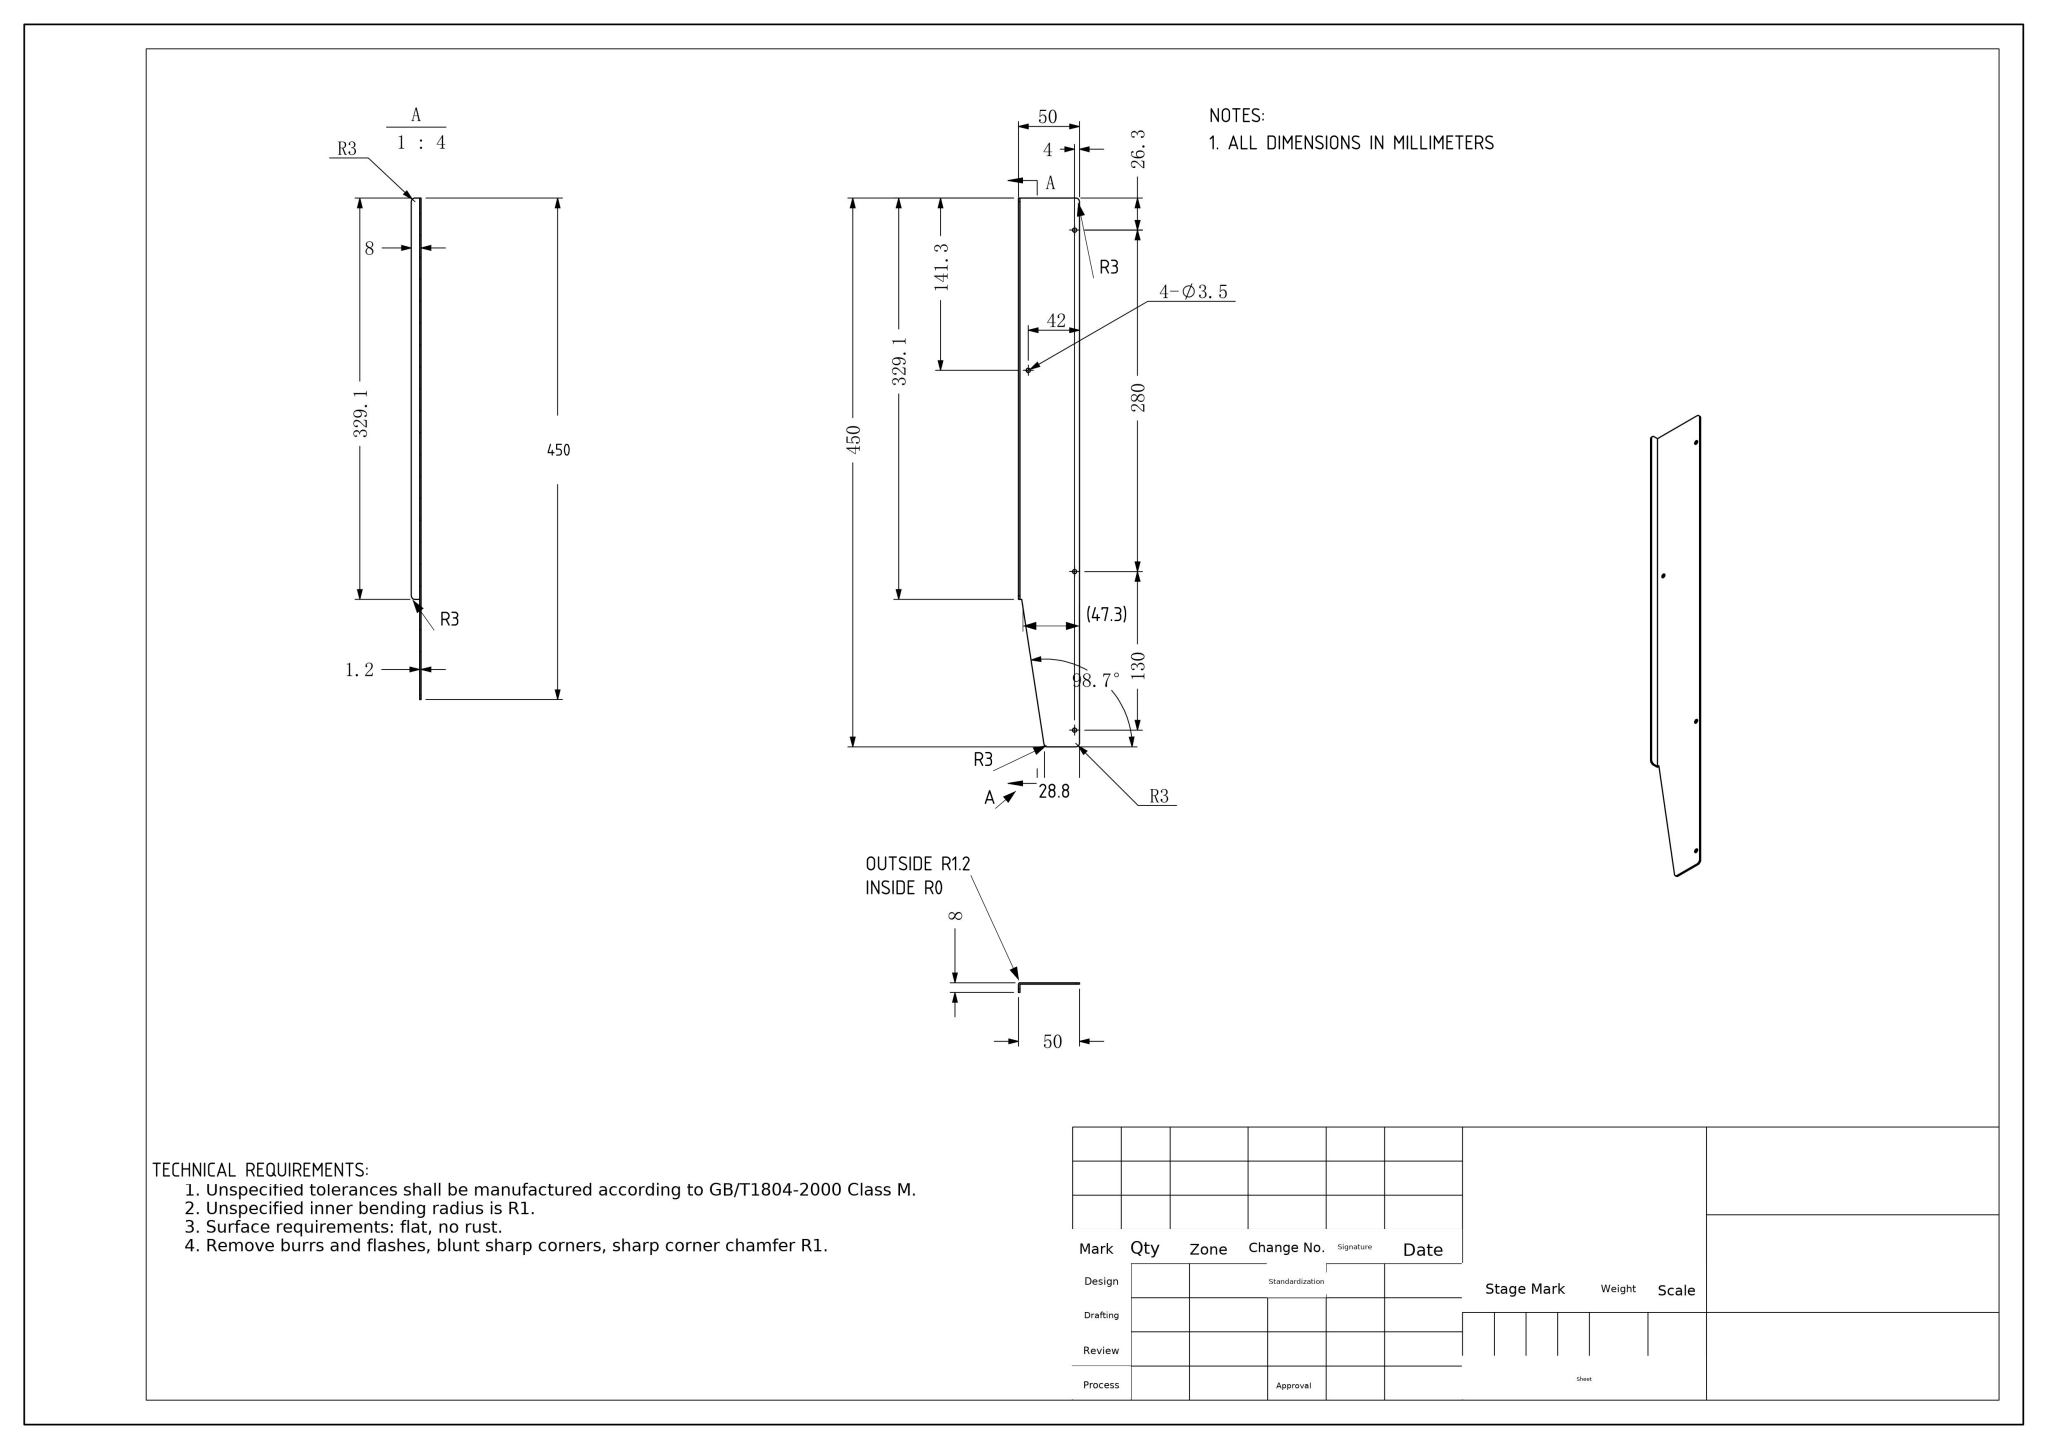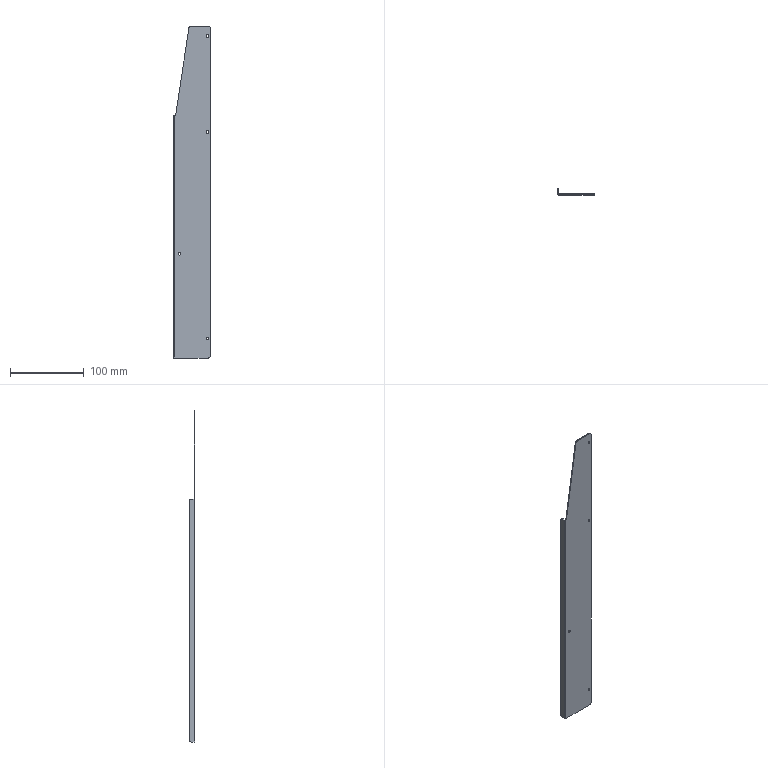Part | NX | mm | Tapered L-Shaped Shelf Bracket 329mm | 1 solid | 25 faces | box 50 x 8 x 450 mm | volume 27790 mm3 | cylinder 15 | plane 10 | commonest cylinder face diameters 3.5 x8 6 x5 2.404 x1 0.004 x1
STEP:
#1=COLOUR_RGB('',0.7529,0.7529,0.7529);
#2=FILL_AREA_STYLE_COLOUR('',#1);
#3=FILL_AREA_STYLE('',(#2));
#4=SURFACE_STYLE_FILL_AREA(#3);
#5=SURFACE_SIDE_STYLE('',(#4));
#6=SURFACE_STYLE_USAGE(.BOTH.,#5);
#7=PRESENTATION_STYLE_ASSIGNMENT((#6));
#8=CARTESIAN_POINT('',(20.,1.2,51.75));
#9=VERTEX_POINT('',#8);
#10=CARTESIAN_POINT('',(20.,1.2,48.25));
#11=VERTEX_POINT('',#10);
#12=CARTESIAN_POINT('',(20.,1.2,50.));
#13=DIRECTION('',(0.,-1.,0.));
#14=DIRECTION('',(0.,0.,-1.));
#15=AXIS2_PLACEMENT_3D('',#12,#13,#14);
#16=CIRCLE('',#15,1.75);
#17=EDGE_CURVE('',#9,#11,#16,.T.);
#18=ORIENTED_EDGE('',*,*,#17,.F.);
#19=CARTESIAN_POINT('',(20.,0.,51.75));
#20=VERTEX_POINT('',#19);
#21=CARTESIAN_POINT('',(20.,0.,51.75));
#22=DIRECTION('',(0.,-1.,0.));
#23=VECTOR('',#22,1000.);
#24=LINE('',#21,#23);
#25=EDGE_CURVE('',#9,#20,#24,.T.);
#26=ORIENTED_EDGE('',*,*,#25,.T.);
#27=CARTESIAN_POINT('',(20.,0.,48.25));
#28=VERTEX_POINT('',#27);
#29=CARTESIAN_POINT('',(20.,0.,50.));
#30=DIRECTION('',(0.,-1.,0.));
#31=DIRECTION('',(0.,0.,-1.));
#32=AXIS2_PLACEMENT_3D('',#29,#30,#31);
#33=CIRCLE('',#32,1.75);
#34=EDGE_CURVE('',#20,#28,#33,.T.);
#35=ORIENTED_EDGE('',*,*,#34,.T.);
#36=CARTESIAN_POINT('',(20.,0.,48.25));
#37=DIRECTION('',(0.,-1.,0.));
#38=VECTOR('',#37,1000.);
#39=LINE('',#36,#38);
#40=EDGE_CURVE('',#11,#28,#39,.T.);
#41=ORIENTED_EDGE('',*,*,#40,.F.);
#42=EDGE_LOOP('',(#18,#26,#35,#41));
#43=FACE_OUTER_BOUND('',#42,.T.);
#44=CARTESIAN_POINT('',(20.,0.,50.));
#45=DIRECTION('',(0.,-1.,0.));
#46=DIRECTION('',(0.,0.,-1.));
#47=AXIS2_PLACEMENT_3D('',#44,#45,#46);
#48=CYLINDRICAL_SURFACE('',#47,1.75);
#49=ADVANCED_FACE('',(#43),#48,.F.);
#50=CARTESIAN_POINT('',(20.,1.2,461.75));
#51=VERTEX_POINT('',#50);
#52=CARTESIAN_POINT('',(20.,1.2,458.25));
#53=VERTEX_POINT('',#52);
#54=CARTESIAN_POINT('',(20.,1.2,460.));
#55=DIRECTION('',(0.,-1.,0.));
#56=DIRECTION('',(0.,0.,-1.));
#57=AXIS2_PLACEMENT_3D('',#54,#55,#56);
#58=CIRCLE('',#57,1.75);
#59=EDGE_CURVE('',#51,#53,#58,.T.);
#60=ORIENTED_EDGE('',*,*,#59,.F.);
#61=CARTESIAN_POINT('',(20.,0.,461.75));
#62=VERTEX_POINT('',#61);
#63=CARTESIAN_POINT('',(20.,0.,461.75));
#64=DIRECTION('',(0.,-1.,0.));
#65=VECTOR('',#64,1000.);
#66=LINE('',#63,#65);
#67=EDGE_CURVE('',#51,#62,#66,.T.);
#68=ORIENTED_EDGE('',*,*,#67,.T.);
#69=CARTESIAN_POINT('',(20.,0.,458.25));
#70=VERTEX_POINT('',#69);
#71=CARTESIAN_POINT('',(20.,0.,460.));
#72=DIRECTION('',(0.,-1.,0.));
#73=DIRECTION('',(0.,0.,-1.));
#74=AXIS2_PLACEMENT_3D('',#71,#72,#73);
#75=CIRCLE('',#74,1.75);
#76=EDGE_CURVE('',#62,#70,#75,.T.);
#77=ORIENTED_EDGE('',*,*,#76,.T.);
#78=CARTESIAN_POINT('',(20.,0.,458.25));
#79=DIRECTION('',(0.,-1.,0.));
#80=VECTOR('',#79,1000.);
#81=LINE('',#78,#80);
#82=EDGE_CURVE('',#53,#70,#81,.T.);
#83=ORIENTED_EDGE('',*,*,#82,.F.);
#84=EDGE_LOOP('',(#60,#68,#77,#83));
#85=FACE_OUTER_BOUND('',#84,.T.);
#86=CARTESIAN_POINT('',(20.,0.,460.));
#87=DIRECTION('',(0.,-1.,0.));
#88=DIRECTION('',(0.,0.,-1.));
#89=AXIS2_PLACEMENT_3D('',#86,#87,#88);
#90=CYLINDRICAL_SURFACE('',#89,1.75);
#91=ADVANCED_FACE('',(#85),#90,.F.);
#92=CARTESIAN_POINT('',(-18.,1.2,163.25));
#93=VERTEX_POINT('',#92);
#94=CARTESIAN_POINT('',(-18.,1.2,166.75));
#95=VERTEX_POINT('',#94);
#96=CARTESIAN_POINT('',(-18.,1.2,165.));
#97=DIRECTION('',(0.,1.,0.));
#98=DIRECTION('',(0.,0.,-1.));
#99=AXIS2_PLACEMENT_3D('',#96,#97,#98);
#100=CIRCLE('',#99,1.75);
#101=EDGE_CURVE('',#93,#95,#100,.T.);
#102=ORIENTED_EDGE('',*,*,#101,.T.);
#103=CARTESIAN_POINT('',(-18.,0.,166.75));
#104=VERTEX_POINT('',#103);
#105=CARTESIAN_POINT('',(-18.,0.,166.75));
#106=DIRECTION('',(0.,-1.,0.));
#107=VECTOR('',#106,1000.);
#108=LINE('',#105,#107);
#109=EDGE_CURVE('',#95,#104,#108,.T.);
#110=ORIENTED_EDGE('',*,*,#109,.T.);
#111=CARTESIAN_POINT('',(-18.,0.,163.25));
#112=VERTEX_POINT('',#111);
#113=CARTESIAN_POINT('',(-18.,0.,165.));
#114=DIRECTION('',(0.,1.,0.));
#115=DIRECTION('',(0.,0.,-1.));
#116=AXIS2_PLACEMENT_3D('',#113,#114,#115);
#117=CIRCLE('',#116,1.75);
#118=EDGE_CURVE('',#112,#104,#117,.T.);
#119=ORIENTED_EDGE('',*,*,#118,.F.);
#120=CARTESIAN_POINT('',(-18.,0.,163.25));
#121=DIRECTION('',(0.,-1.,0.));
#122=VECTOR('',#121,1000.);
#123=LINE('',#120,#122);
#124=EDGE_CURVE('',#93,#112,#123,.T.);
#125=ORIENTED_EDGE('',*,*,#124,.F.);
#126=EDGE_LOOP('',(#102,#110,#119,#125));
#127=FACE_OUTER_BOUND('',#126,.T.);
#128=CARTESIAN_POINT('',(-18.,0.,165.));
#129=DIRECTION('',(0.,-1.,0.));
#130=DIRECTION('',(0.,0.,-1.));
#131=AXIS2_PLACEMENT_3D('',#128,#129,#130);
#132=CYLINDRICAL_SURFACE('',#131,1.75);
#133=ADVANCED_FACE('',(#127),#132,.F.);
#134=CARTESIAN_POINT('',(20.,1.2,331.75));
#135=VERTEX_POINT('',#134);
#136=CARTESIAN_POINT('',(20.,1.2,328.25));
#137=VERTEX_POINT('',#136);
#138=CARTESIAN_POINT('',(20.,1.2,330.));
#139=DIRECTION('',(0.,-1.,0.));
#140=DIRECTION('',(0.,0.,-1.));
#141=AXIS2_PLACEMENT_3D('',#138,#139,#140);
#142=CIRCLE('',#141,1.75);
#143=EDGE_CURVE('',#135,#137,#142,.T.);
#144=ORIENTED_EDGE('',*,*,#143,.F.);
#145=CARTESIAN_POINT('',(20.,0.,331.75));
#146=VERTEX_POINT('',#145);
#147=CARTESIAN_POINT('',(20.,0.,331.75));
#148=DIRECTION('',(0.,-1.,0.));
#149=VECTOR('',#148,1000.);
#150=LINE('',#147,#149);
#151=EDGE_CURVE('',#135,#146,#150,.T.);
#152=ORIENTED_EDGE('',*,*,#151,.T.);
#153=CARTESIAN_POINT('',(20.,0.,328.25));
#154=VERTEX_POINT('',#153);
#155=CARTESIAN_POINT('',(20.,0.,330.));
#156=DIRECTION('',(0.,-1.,0.));
#157=DIRECTION('',(0.,0.,-1.));
#158=AXIS2_PLACEMENT_3D('',#155,#156,#157);
#159=CIRCLE('',#158,1.75);
#160=EDGE_CURVE('',#146,#154,#159,.T.);
#161=ORIENTED_EDGE('',*,*,#160,.T.);
#162=CARTESIAN_POINT('',(20.,0.,328.25));
#163=DIRECTION('',(0.,-1.,0.));
#164=VECTOR('',#163,1000.);
#165=LINE('',#162,#164);
#166=EDGE_CURVE('',#137,#154,#165,.T.);
#167=ORIENTED_EDGE('',*,*,#166,.F.);
#168=EDGE_LOOP('',(#144,#152,#161,#167));
#169=FACE_OUTER_BOUND('',#168,.T.);
#170=CARTESIAN_POINT('',(20.,0.,330.));
#171=DIRECTION('',(0.,-1.,0.));
#172=DIRECTION('',(0.,0.,-1.));
#173=AXIS2_PLACEMENT_3D('',#170,#171,#172);
#174=CYLINDRICAL_SURFACE('',#173,1.75);
#175=ADVANCED_FACE('',(#169),#174,.F.);
#176=CARTESIAN_POINT('',(-24.8,8.,26.703));
#177=VERTEX_POINT('',#176);
#178=CARTESIAN_POINT('',(-24.8,8.,349.8));
#179=VERTEX_POINT('',#178);
#180=CARTESIAN_POINT('',(-24.8,8.,-352.8));
#181=DIRECTION('',(0.,0.,1.));
#182=VECTOR('',#181,1000.);
#183=LINE('',#180,#182);
#184=EDGE_CURVE('',#177,#179,#183,.T.);
#185=ORIENTED_EDGE('',*,*,#184,.F.);
#186=CARTESIAN_POINT('',(-26.,8.,26.703));
#187=VERTEX_POINT('',#186);
#188=CARTESIAN_POINT('',(-25.5,8.,26.703));
#189=DIRECTION('',(-1.,0.,0.));
#190=VECTOR('',#189,1000.);
#191=LINE('',#188,#190);
#192=EDGE_CURVE('',#177,#187,#191,.T.);
#193=ORIENTED_EDGE('',*,*,#192,.T.);
#194=CARTESIAN_POINT('',(-26.,8.,349.8));
#195=VERTEX_POINT('',#194);
#196=CARTESIAN_POINT('',(-26.,8.,-352.8));
#197=DIRECTION('',(0.,0.,1.));
#198=VECTOR('',#197,1000.);
#199=LINE('',#196,#198);
#200=EDGE_CURVE('',#187,#195,#199,.T.);
#201=ORIENTED_EDGE('',*,*,#200,.T.);
#202=CARTESIAN_POINT('',(-25.5,8.,349.8));
#203=DIRECTION('',(1.,0.,0.));
#204=VECTOR('',#203,1000.);
#205=LINE('',#202,#204);
#206=EDGE_CURVE('',#195,#179,#205,.T.);
#207=ORIENTED_EDGE('',*,*,#206,.T.);
#208=EDGE_LOOP('',(#185,#193,#201,#207));
#209=FACE_OUTER_BOUND('',#208,.T.);
#210=CARTESIAN_POINT('',(-25.5,8.,-352.8));
#211=DIRECTION('',(0.,-1.,0.));
#212=DIRECTION('',(0.,0.,1.));
#213=AXIS2_PLACEMENT_3D('',#210,#211,#212);
#214=PLANE('',#213);
#215=ADVANCED_FACE('',(#209),#214,.F.);
#216=CARTESIAN_POINT('',(24.,0.,26.703));
#217=VERTEX_POINT('',#216);
#218=CARTESIAN_POINT('',(24.,0.,470.703));
#219=VERTEX_POINT('',#218);
#220=CARTESIAN_POINT('',(24.,0.,-352.8));
#221=DIRECTION('',(0.,0.,1.));
#222=VECTOR('',#221,1000.);
#223=LINE('',#220,#222);
#224=EDGE_CURVE('',#217,#219,#223,.T.);
#225=ORIENTED_EDGE('',*,*,#224,.F.);
#226=CARTESIAN_POINT('',(24.,1.2,26.703));
#227=VERTEX_POINT('',#226);
#228=CARTESIAN_POINT('',(24.,1.2,26.703));
#229=DIRECTION('',(0.,1.,0.));
#230=VECTOR('',#229,1000.);
#231=LINE('',#228,#230);
#232=EDGE_CURVE('',#217,#227,#231,.T.);
#233=ORIENTED_EDGE('',*,*,#232,.T.);
#234=CARTESIAN_POINT('',(24.,1.2,470.703));
#235=VERTEX_POINT('',#234);
#236=CARTESIAN_POINT('',(24.,1.2,-352.8));
#237=DIRECTION('',(0.,0.,1.));
#238=VECTOR('',#237,1000.);
#239=LINE('',#236,#238);
#240=EDGE_CURVE('',#227,#235,#239,.T.);
#241=ORIENTED_EDGE('',*,*,#240,.T.);
#242=CARTESIAN_POINT('',(24.,0.,470.703));
#243=DIRECTION('',(0.,-1.,0.));
#244=VECTOR('',#243,1000.);
#245=LINE('',#242,#244);
#246=EDGE_CURVE('',#235,#219,#245,.T.);
#247=ORIENTED_EDGE('',*,*,#246,.T.);
#248=EDGE_LOOP('',(#225,#233,#241,#247));
#249=FACE_OUTER_BOUND('',#248,.T.);
#250=CARTESIAN_POINT('',(24.,0.,-352.8));
#251=DIRECTION('',(1.,0.,0.));
#252=DIRECTION('',(0.,0.,1.));
#253=AXIS2_PLACEMENT_3D('',#250,#251,#252);
#254=PLANE('',#253);
#255=ADVANCED_FACE('',(#249),#254,.T.);
#256=CARTESIAN_POINT('',(-24.798,0.,23.703));
#257=VERTEX_POINT('',#256);
#258=CARTESIAN_POINT('',(21.,0.,23.703));
#259=VERTEX_POINT('',#258);
#260=CARTESIAN_POINT('',(-25.5,0.,23.703));
#261=DIRECTION('',(1.,0.,0.));
#262=VECTOR('',#261,1000.);
#263=LINE('',#260,#262);
#264=EDGE_CURVE('',#257,#259,#263,.T.);
#265=ORIENTED_EDGE('',*,*,#264,.T.);
#266=CARTESIAN_POINT('',(21.,0.,26.703));
#267=DIRECTION('',(0.,-1.,0.));
#268=DIRECTION('',(0.,0.,-1.));
#269=AXIS2_PLACEMENT_3D('',#266,#267,#268);
#270=CIRCLE('',#269,3.);
#271=EDGE_CURVE('',#259,#217,#270,.T.);
#272=ORIENTED_EDGE('',*,*,#271,.T.);
#273=ORIENTED_EDGE('',*,*,#224,.T.);
#274=CARTESIAN_POINT('',(21.,0.,473.703));
#275=VERTEX_POINT('',#274);
#276=CARTESIAN_POINT('',(21.,0.,470.703));
#277=DIRECTION('',(0.,-1.,0.));
#278=DIRECTION('',(0.,0.,-1.));
#279=AXIS2_PLACEMENT_3D('',#276,#277,#278);
#280=CIRCLE('',#279,3.);
#281=EDGE_CURVE('',#219,#275,#280,.T.);
#282=ORIENTED_EDGE('',*,*,#281,.T.);
#283=CARTESIAN_POINT('',(-2.188,0.,473.703));
#284=VERTEX_POINT('',#283);
#285=CARTESIAN_POINT('',(24.,0.,473.703));
#286=DIRECTION('',(-1.,0.,0.));
#287=VECTOR('',#286,1000.);
#288=LINE('',#285,#287);
#289=EDGE_CURVE('',#275,#284,#288,.T.);
#290=ORIENTED_EDGE('',*,*,#289,.T.);
#291=CARTESIAN_POINT('',(-5.153,0.,471.158));
#292=VERTEX_POINT('',#291);
#293=CARTESIAN_POINT('',(-2.188,0.,470.703));
#294=DIRECTION('',(0.,-1.,0.));
#295=DIRECTION('',(0.,0.,-1.));
#296=AXIS2_PLACEMENT_3D('',#293,#294,#295);
#297=CIRCLE('',#296,3.);
#298=EDGE_CURVE('',#284,#292,#297,.T.);
#299=ORIENTED_EDGE('',*,*,#298,.T.);
#300=CARTESIAN_POINT('',(-23.298,0.,352.8));
#301=VERTEX_POINT('',#300);
#302=CARTESIAN_POINT('',(-23.298,0.,352.8));
#303=DIRECTION('',(-0.1515,0.,-0.9885));
#304=VECTOR('',#303,1000.);
#305=LINE('',#302,#304);
#306=EDGE_CURVE('',#292,#301,#305,.T.);
#307=ORIENTED_EDGE('',*,*,#306,.T.);
#308=CARTESIAN_POINT('',(-24.798,0.,352.8));
#309=VERTEX_POINT('',#308);
#310=CARTESIAN_POINT('',(-25.5,0.,352.8));
#311=DIRECTION('',(1.,0.,0.));
#312=VECTOR('',#311,1000.);
#313=LINE('',#310,#312);
#314=EDGE_CURVE('',#309,#301,#313,.T.);
#315=ORIENTED_EDGE('',*,*,#314,.F.);
#316=CARTESIAN_POINT('',(-24.798,0.,-352.8));
#317=DIRECTION('',(0.,0.,1.));
#318=VECTOR('',#317,1000.);
#319=LINE('',#316,#318);
#320=EDGE_CURVE('',#257,#309,#319,.T.);
#321=ORIENTED_EDGE('',*,*,#320,.F.);
#322=EDGE_LOOP('',(#265,#272,#273,#282,#290,#299,#307,#315,#321));
#323=FACE_OUTER_BOUND('',#322,.T.);
#324=CARTESIAN_POINT('',(20.,0.,50.));
#325=DIRECTION('',(0.,-1.,0.));
#326=DIRECTION('',(0.,0.,-1.));
#327=AXIS2_PLACEMENT_3D('',#324,#325,#326);
#328=CIRCLE('',#327,1.75);
#329=EDGE_CURVE('',#28,#20,#328,.T.);
#330=ORIENTED_EDGE('',*,*,#329,.F.);
#331=ORIENTED_EDGE('',*,*,#34,.F.);
#332=EDGE_LOOP('',(#330,#331));
#333=FACE_BOUND('',#332,.T.);
#334=CARTESIAN_POINT('',(20.,0.,460.));
#335=DIRECTION('',(0.,-1.,0.));
#336=DIRECTION('',(0.,0.,-1.));
#337=AXIS2_PLACEMENT_3D('',#334,#335,#336);
#338=CIRCLE('',#337,1.75);
#339=EDGE_CURVE('',#70,#62,#338,.T.);
#340=ORIENTED_EDGE('',*,*,#339,.F.);
#341=ORIENTED_EDGE('',*,*,#76,.F.);
#342=EDGE_LOOP('',(#340,#341));
#343=FACE_BOUND('',#342,.T.);
#344=ORIENTED_EDGE('',*,*,#118,.T.);
#345=CARTESIAN_POINT('',(-18.,0.,165.));
#346=DIRECTION('',(0.,1.,0.));
#347=DIRECTION('',(0.,0.,-1.));
#348=AXIS2_PLACEMENT_3D('',#345,#346,#347);
#349=CIRCLE('',#348,1.75);
#350=EDGE_CURVE('',#104,#112,#349,.T.);
#351=ORIENTED_EDGE('',*,*,#350,.T.);
#352=EDGE_LOOP('',(#344,#351));
#353=FACE_BOUND('',#352,.T.);
#354=CARTESIAN_POINT('',(20.,0.,330.));
#355=DIRECTION('',(0.,-1.,0.));
#356=DIRECTION('',(0.,0.,-1.));
#357=AXIS2_PLACEMENT_3D('',#354,#355,#356);
#358=CIRCLE('',#357,1.75);
#359=EDGE_CURVE('',#154,#146,#358,.T.);
#360=ORIENTED_EDGE('',*,*,#359,.F.);
#361=ORIENTED_EDGE('',*,*,#160,.F.);
#362=EDGE_LOOP('',(#360,#361));
#363=FACE_BOUND('',#362,.T.);
#364=CARTESIAN_POINT('',(-25.5,0.,-352.8));
#365=DIRECTION('',(0.,-1.,0.));
#366=DIRECTION('',(0.,0.,-1.));
#367=AXIS2_PLACEMENT_3D('',#364,#365,#366);
#368=PLANE('',#367);
#369=ADVANCED_FACE('',(#323,#333,#343,#353,#363),#368,.T.);
#370=ORIENTED_EDGE('',*,*,#200,.F.);
#371=CARTESIAN_POINT('',(-26.,5.,23.703));
#372=VERTEX_POINT('',#371);
#373=CARTESIAN_POINT('',(-26.,5.,26.703));
#374=DIRECTION('',(-1.,0.,0.));
#375=DIRECTION('',(0.,0.,1.));
#376=AXIS2_PLACEMENT_3D('',#373,#374,#375);
#377=CIRCLE('',#376,3.);
#378=EDGE_CURVE('',#187,#372,#377,.T.);
#379=ORIENTED_EDGE('',*,*,#378,.T.);
#380=CARTESIAN_POINT('',(-26.,1.202,23.703));
#381=VERTEX_POINT('',#380);
#382=CARTESIAN_POINT('',(-26.,8.,23.703));
#383=DIRECTION('',(0.,-1.,0.));
#384=VECTOR('',#383,1000.);
#385=LINE('',#382,#384);
#386=EDGE_CURVE('',#372,#381,#385,.T.);
#387=ORIENTED_EDGE('',*,*,#386,.T.);
#388=CARTESIAN_POINT('',(-26.,1.202,352.8));
#389=VERTEX_POINT('',#388);
#390=CARTESIAN_POINT('',(-26.,1.202,-352.8));
#391=DIRECTION('',(0.,0.,1.));
#392=VECTOR('',#391,1000.);
#393=LINE('',#390,#392);
#394=EDGE_CURVE('',#381,#389,#393,.T.);
#395=ORIENTED_EDGE('',*,*,#394,.T.);
#396=CARTESIAN_POINT('',(-26.,5.,352.8));
#397=VERTEX_POINT('',#396);
#398=CARTESIAN_POINT('',(-26.,8.,352.8));
#399=DIRECTION('',(0.,-1.,0.));
#400=VECTOR('',#399,1000.);
#401=LINE('',#398,#400);
#402=EDGE_CURVE('',#397,#389,#401,.T.);
#403=ORIENTED_EDGE('',*,*,#402,.F.);
#404=CARTESIAN_POINT('',(-26.,5.,349.8));
#405=DIRECTION('',(-1.,0.,0.));
#406=DIRECTION('',(0.,0.,1.));
#407=AXIS2_PLACEMENT_3D('',#404,#405,#406);
#408=CIRCLE('',#407,3.);
#409=EDGE_CURVE('',#397,#195,#408,.T.);
#410=ORIENTED_EDGE('',*,*,#409,.T.);
#411=EDGE_LOOP('',(#370,#379,#387,#395,#403,#410));
#412=FACE_OUTER_BOUND('',#411,.T.);
#413=CARTESIAN_POINT('',(-26.,8.,-352.8));
#414=DIRECTION('',(-1.,0.,0.));
#415=DIRECTION('',(0.,0.,1.));
#416=AXIS2_PLACEMENT_3D('',#413,#414,#415);
#417=PLANE('',#416);
#418=ADVANCED_FACE('',(#412),#417,.T.);
#419=CARTESIAN_POINT('',(-24.798,1.202,23.703));
#420=DIRECTION('',(-0.,0.,1.));
#421=DIRECTION('',(-1.,0.,0.));
#422=AXIS2_PLACEMENT_3D('',#419,#420,#421);
#423=CIRCLE('',#422,1.202);
#424=EDGE_CURVE('',#381,#257,#423,.T.);
#425=ORIENTED_EDGE('',*,*,#424,.T.);
#426=ORIENTED_EDGE('',*,*,#320,.T.);
#427=CARTESIAN_POINT('',(-24.798,1.202,352.8));
#428=DIRECTION('',(0.,0.,1.));
#429=DIRECTION('',(-1.,0.,0.));
#430=AXIS2_PLACEMENT_3D('',#427,#428,#429);
#431=CIRCLE('',#430,1.202);
#432=EDGE_CURVE('',#389,#309,#431,.T.);
#433=ORIENTED_EDGE('',*,*,#432,.F.);
#434=ORIENTED_EDGE('',*,*,#394,.F.);
#435=EDGE_LOOP('',(#425,#426,#433,#434));
#436=FACE_OUTER_BOUND('',#435,.T.);
#437=CARTESIAN_POINT('',(-24.798,1.202,-352.8));
#438=DIRECTION('',(0.,0.,1.));
#439=DIRECTION('',(1.,0.,0.));
#440=AXIS2_PLACEMENT_3D('',#437,#438,#439);
#441=CYLINDRICAL_SURFACE('',#440,1.202);
#442=ADVANCED_FACE('',(#436),#441,.T.);
#443=CARTESIAN_POINT('',(-24.8,5.,352.8));
#444=VERTEX_POINT('',#443);
#445=CARTESIAN_POINT('',(-24.8,1.202,352.8));
#446=VERTEX_POINT('',#445);
#447=CARTESIAN_POINT('',(-24.8,8.,352.8));
#448=DIRECTION('',(0.,-1.,0.));
#449=VECTOR('',#448,1000.);
#450=LINE('',#447,#449);
#451=EDGE_CURVE('',#444,#446,#450,.T.);
#452=ORIENTED_EDGE('',*,*,#451,.F.);
#453=CARTESIAN_POINT('',(-24.298,5.,352.8));
#454=DIRECTION('',(-1.,0.,0.));
#455=VECTOR('',#454,1000.);
#456=LINE('',#453,#455);
#457=EDGE_CURVE('',#444,#397,#456,.T.);
#458=ORIENTED_EDGE('',*,*,#457,.T.);
#459=ORIENTED_EDGE('',*,*,#402,.T.);
#460=ORIENTED_EDGE('',*,*,#432,.T.);
#461=ORIENTED_EDGE('',*,*,#314,.T.);
#462=CARTESIAN_POINT('',(-23.298,1.2,352.8));
#463=VERTEX_POINT('',#462);
#464=CARTESIAN_POINT('',(-23.298,1.2,352.8));
#465=DIRECTION('',(0.,-1.,0.));
#466=VECTOR('',#465,1000.);
#467=LINE('',#464,#466);
#468=EDGE_CURVE('',#463,#301,#467,.T.);
#469=ORIENTED_EDGE('',*,*,#468,.F.);
#470=CARTESIAN_POINT('',(-24.798,1.2,352.8));
#471=VERTEX_POINT('',#470);
#472=CARTESIAN_POINT('',(-25.5,1.2,352.8));
#473=DIRECTION('',(1.,0.,0.));
#474=VECTOR('',#473,1000.);
#475=LINE('',#472,#474);
#476=EDGE_CURVE('',#471,#463,#475,.T.);
#477=ORIENTED_EDGE('',*,*,#476,.F.);
#478=CARTESIAN_POINT('',(-24.798,1.202,352.8));
#479=DIRECTION('',(0.,0.,1.));
#480=DIRECTION('',(1.,0.,0.));
#481=AXIS2_PLACEMENT_3D('',#478,#479,#480);
#482=CIRCLE('',#481,0.002);
#483=EDGE_CURVE('',#446,#471,#482,.T.);
#484=ORIENTED_EDGE('',*,*,#483,.F.);
#485=EDGE_LOOP('',(#452,#458,#459,#460,#461,#469,#477,#484));
#486=FACE_OUTER_BOUND('',#485,.T.);
#487=CARTESIAN_POINT('',(-24.298,1.202,352.8));
#488=DIRECTION('',(0.,0.,1.));
#489=DIRECTION('',(1.,0.,0.));
#490=AXIS2_PLACEMENT_3D('',#487,#488,#489);
#491=PLANE('',#490);
#492=ADVANCED_FACE('',(#486),#491,.T.);
#493=CARTESIAN_POINT('',(20.,1.2,50.));
#494=DIRECTION('',(0.,-1.,0.));
#495=DIRECTION('',(0.,0.,-1.));
#496=AXIS2_PLACEMENT_3D('',#493,#494,#495);
#497=CIRCLE('',#496,1.75);
#498=EDGE_CURVE('',#11,#9,#497,.T.);
#499=ORIENTED_EDGE('',*,*,#498,.T.);
#500=ORIENTED_EDGE('',*,*,#17,.T.);
#501=EDGE_LOOP('',(#499,#500));
#502=FACE_BOUND('',#501,.T.);
#503=CARTESIAN_POINT('',(20.,1.2,460.));
#504=DIRECTION('',(0.,-1.,0.));
#505=DIRECTION('',(0.,0.,-1.));
#506=AXIS2_PLACEMENT_3D('',#503,#504,#505);
#507=CIRCLE('',#506,1.75);
#508=EDGE_CURVE('',#53,#51,#507,.T.);
#509=ORIENTED_EDGE('',*,*,#508,.T.);
#510=ORIENTED_EDGE('',*,*,#59,.T.);
#511=EDGE_LOOP('',(#509,#510));
#512=FACE_BOUND('',#511,.T.);
#513=ORIENTED_EDGE('',*,*,#101,.F.);
#514=CARTESIAN_POINT('',(-18.,1.2,165.));
#515=DIRECTION('',(0.,1.,0.));
#516=DIRECTION('',(0.,0.,-1.));
#517=AXIS2_PLACEMENT_3D('',#514,#515,#516);
#518=CIRCLE('',#517,1.75);
#519=EDGE_CURVE('',#95,#93,#518,.T.);
#520=ORIENTED_EDGE('',*,*,#519,.F.);
#521=EDGE_LOOP('',(#513,#520));
#522=FACE_BOUND('',#521,.T.);
#523=CARTESIAN_POINT('',(20.,1.2,330.));
#524=DIRECTION('',(0.,-1.,0.));
#525=DIRECTION('',(0.,0.,-1.));
#526=AXIS2_PLACEMENT_3D('',#523,#524,#525);
#527=CIRCLE('',#526,1.75);
#528=EDGE_CURVE('',#137,#135,#527,.T.);
#529=ORIENTED_EDGE('',*,*,#528,.T.);
#530=ORIENTED_EDGE('',*,*,#143,.T.);
#531=EDGE_LOOP('',(#529,#530));
#532=FACE_BOUND('',#531,.T.);
#533=ORIENTED_EDGE('',*,*,#240,.F.);
#534=CARTESIAN_POINT('',(21.,1.2,23.703));
#535=VERTEX_POINT('',#534);
#536=CARTESIAN_POINT('',(21.,1.2,26.703));
#537=DIRECTION('',(0.,1.,0.));
#538=DIRECTION('',(0.,0.,-1.));
#539=AXIS2_PLACEMENT_3D('',#536,#537,#538);
#540=CIRCLE('',#539,3.);
#541=EDGE_CURVE('',#227,#535,#540,.T.);
#542=ORIENTED_EDGE('',*,*,#541,.T.);
#543=CARTESIAN_POINT('',(-24.798,1.2,23.703));
#544=VERTEX_POINT('',#543);
#545=CARTESIAN_POINT('',(-25.5,1.2,23.703));
#546=DIRECTION('',(1.,0.,0.));
#547=VECTOR('',#546,1000.);
#548=LINE('',#545,#547);
#549=EDGE_CURVE('',#544,#535,#548,.T.);
#550=ORIENTED_EDGE('',*,*,#549,.F.);
#551=CARTESIAN_POINT('',(-24.798,1.2,-352.8));
#552=DIRECTION('',(0.,0.,1.));
#553=VECTOR('',#552,1000.);
#554=LINE('',#551,#553);
#555=EDGE_CURVE('',#544,#471,#554,.T.);
#556=ORIENTED_EDGE('',*,*,#555,.T.);
#557=ORIENTED_EDGE('',*,*,#476,.T.);
#558=CARTESIAN_POINT('',(-5.153,1.2,471.158));
#559=VERTEX_POINT('',#558);
#560=CARTESIAN_POINT('',(-23.298,1.2,352.8));
#561=DIRECTION('',(-0.1515,0.,-0.9885));
#562=VECTOR('',#561,1000.);
#563=LINE('',#560,#562);
#564=EDGE_CURVE('',#559,#463,#563,.T.);
#565=ORIENTED_EDGE('',*,*,#564,.F.);
#566=CARTESIAN_POINT('',(-2.188,1.2,473.703));
#567=VERTEX_POINT('',#566);
#568=CARTESIAN_POINT('',(-2.188,1.2,470.703));
#569=DIRECTION('',(0.,1.,0.));
#570=DIRECTION('',(0.,0.,-1.));
#571=AXIS2_PLACEMENT_3D('',#568,#569,#570);
#572=CIRCLE('',#571,3.);
#573=EDGE_CURVE('',#559,#567,#572,.T.);
#574=ORIENTED_EDGE('',*,*,#573,.T.);
#575=CARTESIAN_POINT('',(21.,1.2,473.703));
#576=VERTEX_POINT('',#575);
#577=CARTESIAN_POINT('',(24.,1.2,473.703));
#578=DIRECTION('',(-1.,0.,0.));
#579=VECTOR('',#578,1000.);
#580=LINE('',#577,#579);
#581=EDGE_CURVE('',#576,#567,#580,.T.);
#582=ORIENTED_EDGE('',*,*,#581,.F.);
#583=CARTESIAN_POINT('',(21.,1.2,470.703));
#584=DIRECTION('',(0.,1.,0.));
#585=DIRECTION('',(0.,0.,-1.));
#586=AXIS2_PLACEMENT_3D('',#583,#584,#585);
#587=CIRCLE('',#586,3.);
#588=EDGE_CURVE('',#576,#235,#587,.T.);
#589=ORIENTED_EDGE('',*,*,#588,.T.);
#590=EDGE_LOOP('',(#533,#542,#550,#556,#557,#565,#574,#582,#589));
#591=FACE_OUTER_BOUND('',#590,.T.);
#592=CARTESIAN_POINT('',(-25.5,1.2,-352.8));
#593=DIRECTION('',(0.,-1.,0.));
#594=DIRECTION('',(0.,0.,-1.));
#595=AXIS2_PLACEMENT_3D('',#592,#593,#594);
#596=PLANE('',#595);
#597=ADVANCED_FACE('',(#502,#512,#522,#532,#591),#596,.F.);
#598=CARTESIAN_POINT('',(-24.8,5.,23.703));
#599=VERTEX_POINT('',#598);
#600=CARTESIAN_POINT('',(-24.8,1.202,23.703));
#601=VERTEX_POINT('',#600);
#602=CARTESIAN_POINT('',(-24.8,8.,23.703));
#603=DIRECTION('',(0.,-1.,0.));
#604=VECTOR('',#603,1000.);
#605=LINE('',#602,#604);
#606=EDGE_CURVE('',#599,#601,#605,.T.);
#607=ORIENTED_EDGE('',*,*,#606,.F.);
#608=CARTESIAN_POINT('',(-24.8,5.,26.703));
#609=DIRECTION('',(1.,0.,0.));
#610=DIRECTION('',(0.,0.,1.));
#611=AXIS2_PLACEMENT_3D('',#608,#609,#610);
#612=CIRCLE('',#611,3.);
#613=EDGE_CURVE('',#599,#177,#612,.T.);
#614=ORIENTED_EDGE('',*,*,#613,.T.);
#615=ORIENTED_EDGE('',*,*,#184,.T.);
#616=CARTESIAN_POINT('',(-24.8,5.,349.8));
#617=DIRECTION('',(1.,0.,0.));
#618=DIRECTION('',(0.,0.,1.));
#619=AXIS2_PLACEMENT_3D('',#616,#617,#618);
#620=CIRCLE('',#619,3.);
#621=EDGE_CURVE('',#179,#444,#620,.T.);
#622=ORIENTED_EDGE('',*,*,#621,.T.);
#623=ORIENTED_EDGE('',*,*,#451,.T.);
#624=CARTESIAN_POINT('',(-24.8,1.202,-352.8));
#625=DIRECTION('',(0.,0.,1.));
#626=VECTOR('',#625,1000.);
#627=LINE('',#624,#626);
#628=EDGE_CURVE('',#601,#446,#627,.T.);
#629=ORIENTED_EDGE('',*,*,#628,.F.);
#630=EDGE_LOOP('',(#607,#614,#615,#622,#623,#629));
#631=FACE_OUTER_BOUND('',#630,.T.);
#632=CARTESIAN_POINT('',(-24.8,8.,-352.8));
#633=DIRECTION('',(-1.,0.,0.));
#634=DIRECTION('',(0.,0.,1.));
#635=AXIS2_PLACEMENT_3D('',#632,#633,#634);
#636=PLANE('',#635);
#637=ADVANCED_FACE('',(#631),#636,.F.);
#638=ORIENTED_EDGE('',*,*,#555,.F.);
#639=CARTESIAN_POINT('',(-24.798,1.202,23.703));
#640=DIRECTION('',(0.,0.,1.));
#641=DIRECTION('',(1.,0.,0.));
#642=AXIS2_PLACEMENT_3D('',#639,#640,#641);
#643=CIRCLE('',#642,0.002);
#644=EDGE_CURVE('',#601,#544,#643,.T.);
#645=ORIENTED_EDGE('',*,*,#644,.F.);
#646=ORIENTED_EDGE('',*,*,#628,.T.);
#647=ORIENTED_EDGE('',*,*,#483,.T.);
#648=EDGE_LOOP('',(#638,#645,#646,#647));
#649=FACE_OUTER_BOUND('',#648,.T.);
#650=CARTESIAN_POINT('',(-24.798,1.202,-352.8));
#651=DIRECTION('',(0.,0.,1.));
#652=DIRECTION('',(1.,0.,0.));
#653=AXIS2_PLACEMENT_3D('',#650,#651,#652);
#654=CYLINDRICAL_SURFACE('',#653,0.002);
#655=ADVANCED_FACE('',(#649),#654,.F.);
#656=ORIENTED_EDGE('',*,*,#306,.F.);
#657=CARTESIAN_POINT('',(-5.153,1.2,471.158));
#658=DIRECTION('',(0.,1.,0.));
#659=VECTOR('',#658,1000.);
#660=LINE('',#657,#659);
#661=EDGE_CURVE('',#292,#559,#660,.T.);
#662=ORIENTED_EDGE('',*,*,#661,.T.);
#663=ORIENTED_EDGE('',*,*,#564,.T.);
#664=ORIENTED_EDGE('',*,*,#468,.T.);
#665=EDGE_LOOP('',(#656,#662,#663,#664));
#666=FACE_OUTER_BOUND('',#665,.T.);
#667=CARTESIAN_POINT('',(-23.298,1.2,352.8));
#668=DIRECTION('',(-0.9885,0.,0.1515));
#669=DIRECTION('',(0.1515,0.,0.9885));
#670=AXIS2_PLACEMENT_3D('',#667,#668,#669);
#671=PLANE('',#670);
#672=ADVANCED_FACE('',(#666),#671,.T.);
#673=ORIENTED_EDGE('',*,*,#581,.T.);
#674=CARTESIAN_POINT('',(-2.188,1.2,473.703));
#675=DIRECTION('',(0.,-1.,0.));
#676=VECTOR('',#675,1000.);
#677=LINE('',#674,#676);
#678=EDGE_CURVE('',#567,#284,#677,.T.);
#679=ORIENTED_EDGE('',*,*,#678,.T.);
#680=ORIENTED_EDGE('',*,*,#289,.F.);
#681=CARTESIAN_POINT('',(21.,1.2,473.703));
#682=DIRECTION('',(0.,1.,0.));
#683=VECTOR('',#682,1000.);
#684=LINE('',#681,#683);
#685=EDGE_CURVE('',#275,#576,#684,.T.);
#686=ORIENTED_EDGE('',*,*,#685,.T.);
#687=EDGE_LOOP('',(#673,#679,#680,#686));
#688=FACE_OUTER_BOUND('',#687,.T.);
#689=CARTESIAN_POINT('',(24.,1.2,473.703));
#690=DIRECTION('',(0.,0.,1.));
#691=DIRECTION('',(1.,0.,0.));
#692=AXIS2_PLACEMENT_3D('',#689,#690,#691);
#693=PLANE('',#692);
#694=ADVANCED_FACE('',(#688),#693,.T.);
#695=ORIENTED_EDGE('',*,*,#151,.F.);
#696=ORIENTED_EDGE('',*,*,#528,.F.);
#697=ORIENTED_EDGE('',*,*,#166,.T.);
#698=ORIENTED_EDGE('',*,*,#359,.T.);
#699=EDGE_LOOP('',(#695,#696,#697,#698));
#700=FACE_OUTER_BOUND('',#699,.T.);
#701=CARTESIAN_POINT('',(20.,0.,330.));
#702=DIRECTION('',(0.,-1.,0.));
#703=DIRECTION('',(0.,0.,-1.));
#704=AXIS2_PLACEMENT_3D('',#701,#702,#703);
#705=CYLINDRICAL_SURFACE('',#704,1.75);
#706=ADVANCED_FACE('',(#700),#705,.F.);
#707=ORIENTED_EDGE('',*,*,#109,.F.);
#708=ORIENTED_EDGE('',*,*,#519,.T.);
#709=ORIENTED_EDGE('',*,*,#124,.T.);
#710=ORIENTED_EDGE('',*,*,#350,.F.);
#711=EDGE_LOOP('',(#707,#708,#709,#710));
#712=FACE_OUTER_BOUND('',#711,.T.);
#713=CARTESIAN_POINT('',(-18.,0.,165.));
#714=DIRECTION('',(0.,-1.,0.));
#715=DIRECTION('',(0.,0.,-1.));
#716=AXIS2_PLACEMENT_3D('',#713,#714,#715);
#717=CYLINDRICAL_SURFACE('',#716,1.75);
#718=ADVANCED_FACE('',(#712),#717,.F.);
#719=ORIENTED_EDGE('',*,*,#67,.F.);
#720=ORIENTED_EDGE('',*,*,#508,.F.);
#721=ORIENTED_EDGE('',*,*,#82,.T.);
#722=ORIENTED_EDGE('',*,*,#339,.T.);
#723=EDGE_LOOP('',(#719,#720,#721,#722));
#724=FACE_OUTER_BOUND('',#723,.T.);
#725=CARTESIAN_POINT('',(20.,0.,460.));
#726=DIRECTION('',(0.,-1.,0.));
#727=DIRECTION('',(0.,0.,-1.));
#728=AXIS2_PLACEMENT_3D('',#725,#726,#727);
#729=CYLINDRICAL_SURFACE('',#728,1.75);
#730=ADVANCED_FACE('',(#724),#729,.F.);
#731=ORIENTED_EDGE('',*,*,#25,.F.);
#732=ORIENTED_EDGE('',*,*,#498,.F.);
#733=ORIENTED_EDGE('',*,*,#40,.T.);
#734=ORIENTED_EDGE('',*,*,#329,.T.);
#735=EDGE_LOOP('',(#731,#732,#733,#734));
#736=FACE_OUTER_BOUND('',#735,.T.);
#737=CARTESIAN_POINT('',(20.,0.,50.));
#738=DIRECTION('',(0.,-1.,0.));
#739=DIRECTION('',(0.,0.,-1.));
#740=AXIS2_PLACEMENT_3D('',#737,#738,#739);
#741=CYLINDRICAL_SURFACE('',#740,1.75);
#742=ADVANCED_FACE('',(#736),#741,.F.);
#743=ORIENTED_EDGE('',*,*,#621,.F.);
#744=ORIENTED_EDGE('',*,*,#206,.F.);
#745=ORIENTED_EDGE('',*,*,#409,.F.);
#746=ORIENTED_EDGE('',*,*,#457,.F.);
#747=EDGE_LOOP('',(#743,#744,#745,#746));
#748=FACE_OUTER_BOUND('',#747,.T.);
#749=CARTESIAN_POINT('',(-24.298,5.,349.8));
#750=DIRECTION('',(1.,0.,0.));
#751=DIRECTION('',(0.,0.,-1.));
#752=AXIS2_PLACEMENT_3D('',#749,#750,#751);
#753=CYLINDRICAL_SURFACE('',#752,3.);
#754=ADVANCED_FACE('',(#748),#753,.T.);
#755=ORIENTED_EDGE('',*,*,#573,.F.);
#756=ORIENTED_EDGE('',*,*,#661,.F.);
#757=ORIENTED_EDGE('',*,*,#298,.F.);
#758=ORIENTED_EDGE('',*,*,#678,.F.);
#759=EDGE_LOOP('',(#755,#756,#757,#758));
#760=FACE_OUTER_BOUND('',#759,.T.);
#761=CARTESIAN_POINT('',(-2.188,1.2,470.703));
#762=DIRECTION('',(0.,-1.,0.));
#763=DIRECTION('',(0.,0.,-1.));
#764=AXIS2_PLACEMENT_3D('',#761,#762,#763);
#765=CYLINDRICAL_SURFACE('',#764,3.);
#766=ADVANCED_FACE('',(#760),#765,.T.);
#767=ORIENTED_EDGE('',*,*,#588,.F.);
#768=ORIENTED_EDGE('',*,*,#685,.F.);
#769=ORIENTED_EDGE('',*,*,#281,.F.);
#770=ORIENTED_EDGE('',*,*,#246,.F.);
#771=EDGE_LOOP('',(#767,#768,#769,#770));
#772=FACE_OUTER_BOUND('',#771,.T.);
#773=CARTESIAN_POINT('',(21.,0.,470.703));
#774=DIRECTION('',(0.,-1.,0.));
#775=DIRECTION('',(0.,0.,-1.));
#776=AXIS2_PLACEMENT_3D('',#773,#774,#775);
#777=CYLINDRICAL_SURFACE('',#776,3.);
#778=ADVANCED_FACE('',(#772),#777,.T.);
#779=ORIENTED_EDGE('',*,*,#386,.F.);
#780=CARTESIAN_POINT('',(-24.3,5.,23.703));
#781=DIRECTION('',(1.,0.,0.));
#782=VECTOR('',#781,1000.);
#783=LINE('',#780,#782);
#784=EDGE_CURVE('',#372,#599,#783,.T.);
#785=ORIENTED_EDGE('',*,*,#784,.T.);
#786=ORIENTED_EDGE('',*,*,#606,.T.);
#787=ORIENTED_EDGE('',*,*,#644,.T.);
#788=ORIENTED_EDGE('',*,*,#549,.T.);
#789=CARTESIAN_POINT('',(21.,0.,23.703));
#790=DIRECTION('',(0.,-1.,0.));
#791=VECTOR('',#790,1000.);
#792=LINE('',#789,#791);
#793=EDGE_CURVE('',#535,#259,#792,.T.);
#794=ORIENTED_EDGE('',*,*,#793,.T.);
#795=ORIENTED_EDGE('',*,*,#264,.F.);
#796=ORIENTED_EDGE('',*,*,#424,.F.);
#797=EDGE_LOOP('',(#779,#785,#786,#787,#788,#794,#795,#796));
#798=FACE_OUTER_BOUND('',#797,.T.);
#799=CARTESIAN_POINT('',(-25.5,8.,23.703));
#800=DIRECTION('',(0.,0.,-1.));
#801=DIRECTION('',(0.,-1.,0.));
#802=AXIS2_PLACEMENT_3D('',#799,#800,#801);
#803=PLANE('',#802);
#804=ADVANCED_FACE('',(#798),#803,.T.);
#805=ORIENTED_EDGE('',*,*,#613,.F.);
#806=ORIENTED_EDGE('',*,*,#784,.F.);
#807=ORIENTED_EDGE('',*,*,#378,.F.);
#808=ORIENTED_EDGE('',*,*,#192,.F.);
#809=EDGE_LOOP('',(#805,#806,#807,#808));
#810=FACE_OUTER_BOUND('',#809,.T.);
#811=CARTESIAN_POINT('',(-25.5,5.,26.703));
#812=DIRECTION('',(1.,0.,0.));
#813=DIRECTION('',(0.,0.,-1.));
#814=AXIS2_PLACEMENT_3D('',#811,#812,#813);
#815=CYLINDRICAL_SURFACE('',#814,3.);
#816=ADVANCED_FACE('',(#810),#815,.T.);
#817=ORIENTED_EDGE('',*,*,#541,.F.);
#818=ORIENTED_EDGE('',*,*,#232,.F.);
#819=ORIENTED_EDGE('',*,*,#271,.F.);
#820=ORIENTED_EDGE('',*,*,#793,.F.);
#821=EDGE_LOOP('',(#817,#818,#819,#820));
#822=FACE_OUTER_BOUND('',#821,.T.);
#823=CARTESIAN_POINT('',(21.,8.,26.703));
#824=DIRECTION('',(0.,-1.,0.));
#825=DIRECTION('',(0.,0.,-1.));
#826=AXIS2_PLACEMENT_3D('',#823,#824,#825);
#827=CYLINDRICAL_SURFACE('',#826,3.);
#828=ADVANCED_FACE('',(#822),#827,.T.);
#829=CLOSED_SHELL('',(#49,#91,#133,#175,#215,#255,#369,#418,#442,#492,#597,#637,#655,#672,#694,#706,#718,#730,#742,#754,#766,#778,#804,#816,#828));
#830=MANIFOLD_SOLID_BREP('',#829);
#831=CARTESIAN_POINT('',(0.,0.,0.));
#832=DIRECTION('',(0.,0.,1.));
#833=DIRECTION('',(1.,0.,0.));
#834=AXIS2_PLACEMENT_3D('',#831,#832,#833);
#835=(LENGTH_UNIT()NAMED_UNIT(*)SI_UNIT(.MILLI.,.METRE.));
#836=UNCERTAINTY_MEASURE_WITH_UNIT(LENGTH_MEASURE(0.00001),#835,'','');
#837=(NAMED_UNIT(*)PLANE_ANGLE_UNIT()SI_UNIT($,.RADIAN.));
#838=(NAMED_UNIT(*)SI_UNIT($,.STERADIAN.)SOLID_ANGLE_UNIT());
#839=(GEOMETRIC_REPRESENTATION_CONTEXT(3)GLOBAL_UNCERTAINTY_ASSIGNED_CONTEXT((#836))GLOBAL_UNIT_ASSIGNED_CONTEXT((#835,#837,#838))REPRESENTATION_CONTEXT('',''));
#840=ADVANCED_BREP_SHAPE_REPRESENTATION('',(#830,#834),#839);
#841=STYLED_ITEM('',(#7),#840);
#842=(LENGTH_UNIT()NAMED_UNIT(*)SI_UNIT(.MILLI.,.METRE.));
#843=UNCERTAINTY_MEASURE_WITH_UNIT(LENGTH_MEASURE(0.00001),#842,'','');
#844=(NAMED_UNIT(*)PLANE_ANGLE_UNIT()SI_UNIT($,.RADIAN.));
#845=(NAMED_UNIT(*)SI_UNIT($,.STERADIAN.)SOLID_ANGLE_UNIT());
#846=(GEOMETRIC_REPRESENTATION_CONTEXT(3)GLOBAL_UNCERTAINTY_ASSIGNED_CONTEXT((#843))GLOBAL_UNIT_ASSIGNED_CONTEXT((#842,#844,#845))REPRESENTATION_CONTEXT('',''));
#847=MECHANICAL_DESIGN_GEOMETRIC_PRESENTATION_REPRESENTATION('',(#841),#846);
#848=COLOUR_RGB('',0.7529,0.7529,0.7529);
#849=FILL_AREA_STYLE_COLOUR('',#848);
#850=FILL_AREA_STYLE('',(#849));
#851=SURFACE_STYLE_FILL_AREA(#850);
#852=SURFACE_SIDE_STYLE('',(#851));
#853=SURFACE_STYLE_USAGE(.BOTH.,#852);
#854=PRESENTATION_STYLE_ASSIGNMENT((#853));
#855=STYLED_ITEM('',(#854),#830);
#856=(LENGTH_UNIT()NAMED_UNIT(*)SI_UNIT(.MILLI.,.METRE.));
#857=UNCERTAINTY_MEASURE_WITH_UNIT(LENGTH_MEASURE(0.00001),#856,'','');
#858=(NAMED_UNIT(*)PLANE_ANGLE_UNIT()SI_UNIT($,.RADIAN.));
#859=(NAMED_UNIT(*)SI_UNIT($,.STERADIAN.)SOLID_ANGLE_UNIT());
#860=(GEOMETRIC_REPRESENTATION_CONTEXT(3)GLOBAL_UNCERTAINTY_ASSIGNED_CONTEXT((#857))GLOBAL_UNIT_ASSIGNED_CONTEXT((#856,#858,#859))REPRESENTATION_CONTEXT('',''));
#861=MECHANICAL_DESIGN_GEOMETRIC_PRESENTATION_REPRESENTATION('',(#855),#860);
#862=PRESENTATION_LAYER_ASSIGNMENT('','',(#855));
#863=PRESENTATION_LAYER_ASSIGNMENT('','',(#841));